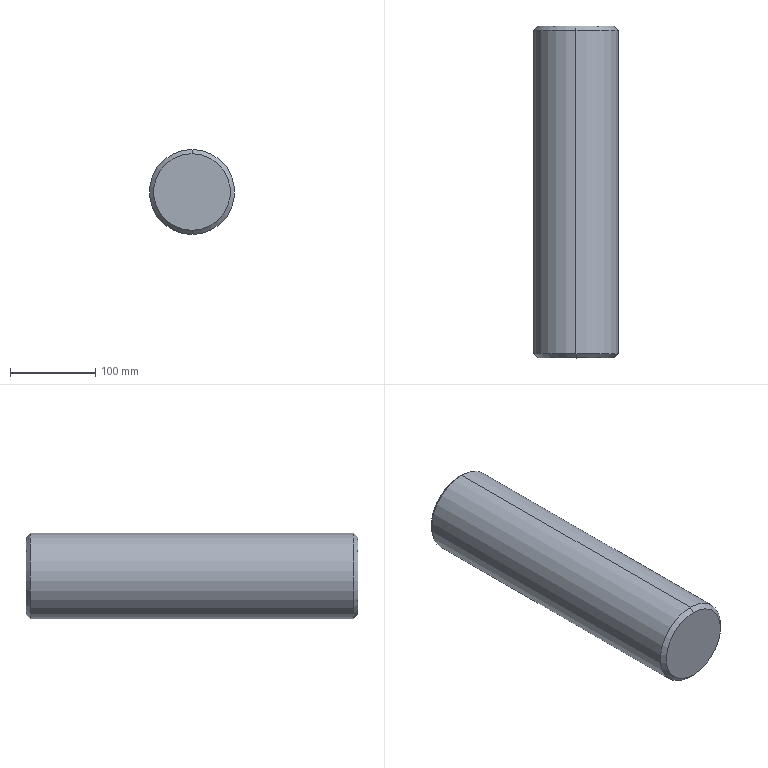Component | SolidWorks | Axis-1 | 1 solid | 8 faces | box 100 x 390 x 100 mm | volume 3055461 mm3 | cone 4 | cylinder 2 | plane 2 | commonest cylinder face diameters 100 x2 | material Plain Carbon Steel
build123d program:
from build123d import *

# Parameters (mm, degrees)
SKETCH1_R           = 50
BOSS_EXTRUDE1_DEPTH = 390
CHAMFER1_SIZE       = 5


with BuildPart() as part:
    # Sketch1 → Boss-Extrude1 (new body)
    with BuildSketch(Plane(origin=(0, 0, 0), x_dir=(0, 0, -1), z_dir=(1, 0, 0))):
        Circle(SKETCH1_R)
    extrude(amount=BOSS_EXTRUDE1_DEPTH)

    # Chamfer1
    chamfer1_edges = [part.edges().sort_by_distance(p)[0] for p in [
        (0, 0, 50),
        (390, 0, 50),
    ]]
    chamfer(chamfer1_edges, length=CHAMFER1_SIZE)


solid = part.part

# Placed as in the assembly
solid = solid.moved(Location((1250.579, 1061.349, 1853.088), (0, 0, 90)))
STEP:
#1=COLOUR_RGB('',0.7922,0.8196,0.9333);
#2=FILL_AREA_STYLE_COLOUR('',#1);
#3=FILL_AREA_STYLE('',(#2));
#4=SURFACE_STYLE_FILL_AREA(#3);
#5=SURFACE_SIDE_STYLE('',(#4));
#6=SURFACE_STYLE_USAGE(.BOTH.,#5);
#7=PRESENTATION_STYLE_ASSIGNMENT((#6));
#8=CARTESIAN_POINT('',(49.235,41.785,74.728));
#9=VERTEX_POINT('',#8);
#10=CARTESIAN_POINT('',(49.235,41.785,71.185));
#11=VERTEX_POINT('',#10);
#12=CARTESIAN_POINT('',(49.235,41.785,72.956));
#13=DIRECTION('',(0.,-1.,0.));
#14=DIRECTION('',(0.,0.,-1.));
#15=AXIS2_PLACEMENT_3D('',#12,#13,#14);
#16=CIRCLE('',#15,1.772);
#17=EDGE_CURVE('',#9,#11,#16,.T.);
#18=ORIENTED_EDGE('',*,*,#17,.F.);
#19=CARTESIAN_POINT('',(49.235,41.982,74.925));
#20=VERTEX_POINT('',#19);
#21=CARTESIAN_POINT('',(49.235,41.982,74.925));
#22=DIRECTION('',(-0.,0.7071,0.7071));
#23=VECTOR('',#22,39.37);
#24=LINE('',#21,#23);
#25=EDGE_CURVE('',#9,#20,#24,.T.);
#26=ORIENTED_EDGE('',*,*,#25,.T.);
#27=CARTESIAN_POINT('',(49.235,41.982,70.988));
#28=VERTEX_POINT('',#27);
#29=CARTESIAN_POINT('',(49.235,41.982,72.956));
#30=DIRECTION('',(-0.,1.,0.));
#31=DIRECTION('',(0.,0.,-1.));
#32=AXIS2_PLACEMENT_3D('',#29,#30,#31);
#33=CIRCLE('',#32,1.969);
#34=EDGE_CURVE('',#28,#20,#33,.T.);
#35=ORIENTED_EDGE('',*,*,#34,.F.);
#36=CARTESIAN_POINT('',(49.235,41.982,70.988));
#37=DIRECTION('',(-0.,0.7071,-0.7071));
#38=VECTOR('',#37,39.37);
#39=LINE('',#36,#38);
#40=EDGE_CURVE('',#11,#28,#39,.T.);
#41=ORIENTED_EDGE('',*,*,#40,.F.);
#42=EDGE_LOOP('',(#18,#26,#35,#41));
#43=FACE_OUTER_BOUND('',#42,.T.);
#44=CARTESIAN_POINT('',(49.235,41.982,72.956));
#45=DIRECTION('',(-0.,1.,0.));
#46=DIRECTION('',(0.,0.,-1.));
#47=AXIS2_PLACEMENT_3D('',#44,#45,#46);
#48=CONICAL_SURFACE('',#47,1.969,0.7854);
#49=ADVANCED_FACE('',(#43),#48,.T.);
#50=CARTESIAN_POINT('',(49.235,57.14,71.185));
#51=VERTEX_POINT('',#50);
#52=CARTESIAN_POINT('',(49.235,57.14,74.728));
#53=VERTEX_POINT('',#52);
#54=CARTESIAN_POINT('',(49.235,57.14,72.956));
#55=DIRECTION('',(-0.,1.,0.));
#56=DIRECTION('',(0.,0.,-1.));
#57=AXIS2_PLACEMENT_3D('',#54,#55,#56);
#58=CIRCLE('',#57,1.772);
#59=EDGE_CURVE('',#51,#53,#58,.T.);
#60=ORIENTED_EDGE('',*,*,#59,.F.);
#61=CARTESIAN_POINT('',(49.235,56.943,70.988));
#62=VERTEX_POINT('',#61);
#63=CARTESIAN_POINT('',(49.235,57.14,71.185));
#64=DIRECTION('',(0.,-0.7071,-0.7071));
#65=VECTOR('',#64,39.37);
#66=LINE('',#63,#65);
#67=EDGE_CURVE('',#51,#62,#66,.T.);
#68=ORIENTED_EDGE('',*,*,#67,.T.);
#69=CARTESIAN_POINT('',(49.235,56.943,74.925));
#70=VERTEX_POINT('',#69);
#71=CARTESIAN_POINT('',(49.235,56.943,72.956));
#72=DIRECTION('',(0.,-1.,0.));
#73=DIRECTION('',(-0.,0.,-1.));
#74=AXIS2_PLACEMENT_3D('',#71,#72,#73);
#75=CIRCLE('',#74,1.969);
#76=EDGE_CURVE('',#70,#62,#75,.T.);
#77=ORIENTED_EDGE('',*,*,#76,.F.);
#78=CARTESIAN_POINT('',(49.235,57.14,74.728));
#79=DIRECTION('',(0.,-0.7071,0.7071));
#80=VECTOR('',#79,39.37);
#81=LINE('',#78,#80);
#82=EDGE_CURVE('',#53,#70,#81,.T.);
#83=ORIENTED_EDGE('',*,*,#82,.F.);
#84=EDGE_LOOP('',(#60,#68,#77,#83));
#85=FACE_OUTER_BOUND('',#84,.T.);
#86=CARTESIAN_POINT('',(49.235,57.14,72.956));
#87=DIRECTION('',(0.,-1.,0.));
#88=DIRECTION('',(0.,0.,1.));
#89=AXIS2_PLACEMENT_3D('',#86,#87,#88);
#90=CONICAL_SURFACE('',#89,1.772,0.7854);
#91=ADVANCED_FACE('',(#85),#90,.T.);
#92=ORIENTED_EDGE('',*,*,#76,.T.);
#93=CARTESIAN_POINT('',(49.235,57.14,70.988));
#94=DIRECTION('',(0.,-1.,0.));
#95=VECTOR('',#94,39.37);
#96=LINE('',#93,#95);
#97=EDGE_CURVE('',#62,#28,#96,.T.);
#98=ORIENTED_EDGE('',*,*,#97,.T.);
#99=ORIENTED_EDGE('',*,*,#34,.T.);
#100=CARTESIAN_POINT('',(49.235,57.14,74.925));
#101=DIRECTION('',(0.,-1.,0.));
#102=VECTOR('',#101,39.37);
#103=LINE('',#100,#102);
#104=EDGE_CURVE('',#70,#20,#103,.T.);
#105=ORIENTED_EDGE('',*,*,#104,.F.);
#106=EDGE_LOOP('',(#92,#98,#99,#105));
#107=FACE_OUTER_BOUND('',#106,.T.);
#108=CARTESIAN_POINT('',(49.235,57.14,72.956));
#109=DIRECTION('',(0.,-1.,0.));
#110=DIRECTION('',(0.,0.,1.));
#111=AXIS2_PLACEMENT_3D('',#108,#109,#110);
#112=CYLINDRICAL_SURFACE('',#111,1.969);
#113=ADVANCED_FACE('',(#107),#112,.T.);
#114=ORIENTED_EDGE('',*,*,#97,.F.);
#115=CARTESIAN_POINT('',(49.235,56.943,72.956));
#116=DIRECTION('',(0.,-1.,0.));
#117=DIRECTION('',(0.,0.,-1.));
#118=AXIS2_PLACEMENT_3D('',#115,#116,#117);
#119=CIRCLE('',#118,1.969);
#120=EDGE_CURVE('',#62,#70,#119,.T.);
#121=ORIENTED_EDGE('',*,*,#120,.T.);
#122=ORIENTED_EDGE('',*,*,#104,.T.);
#123=CARTESIAN_POINT('',(49.235,41.982,72.956));
#124=DIRECTION('',(-0.,1.,0.));
#125=DIRECTION('',(0.,0.,-1.));
#126=AXIS2_PLACEMENT_3D('',#123,#124,#125);
#127=CIRCLE('',#126,1.969);
#128=EDGE_CURVE('',#20,#28,#127,.T.);
#129=ORIENTED_EDGE('',*,*,#128,.T.);
#130=EDGE_LOOP('',(#114,#121,#122,#129));
#131=FACE_OUTER_BOUND('',#130,.T.);
#132=CARTESIAN_POINT('',(49.235,57.14,72.956));
#133=DIRECTION('',(0.,-1.,0.));
#134=DIRECTION('',(0.,0.,1.));
#135=AXIS2_PLACEMENT_3D('',#132,#133,#134);
#136=CYLINDRICAL_SURFACE('',#135,1.969);
#137=ADVANCED_FACE('',(#131),#136,.T.);
#138=CARTESIAN_POINT('',(49.235,57.14,72.956));
#139=DIRECTION('',(-0.,1.,0.));
#140=DIRECTION('',(0.,0.,-1.));
#141=AXIS2_PLACEMENT_3D('',#138,#139,#140);
#142=CIRCLE('',#141,1.772);
#143=EDGE_CURVE('',#53,#51,#142,.T.);
#144=ORIENTED_EDGE('',*,*,#143,.T.);
#145=ORIENTED_EDGE('',*,*,#59,.T.);
#146=EDGE_LOOP('',(#144,#145));
#147=FACE_OUTER_BOUND('',#146,.T.);
#148=CARTESIAN_POINT('',(49.235,57.14,72.956));
#149=DIRECTION('',(-0.,1.,0.));
#150=DIRECTION('',(0.,0.,-1.));
#151=AXIS2_PLACEMENT_3D('',#148,#149,#150);
#152=PLANE('',#151);
#153=ADVANCED_FACE('',(#147),#152,.T.);
#154=CARTESIAN_POINT('',(49.235,41.785,72.956));
#155=DIRECTION('',(0.,-1.,0.));
#156=DIRECTION('',(0.,0.,-1.));
#157=AXIS2_PLACEMENT_3D('',#154,#155,#156);
#158=CIRCLE('',#157,1.772);
#159=EDGE_CURVE('',#11,#9,#158,.T.);
#160=ORIENTED_EDGE('',*,*,#159,.T.);
#161=ORIENTED_EDGE('',*,*,#17,.T.);
#162=EDGE_LOOP('',(#160,#161));
#163=FACE_OUTER_BOUND('',#162,.T.);
#164=CARTESIAN_POINT('',(49.235,41.785,72.956));
#165=DIRECTION('',(-0.,1.,0.));
#166=DIRECTION('',(0.,0.,-1.));
#167=AXIS2_PLACEMENT_3D('',#164,#165,#166);
#168=PLANE('',#167);
#169=ADVANCED_FACE('',(#163),#168,.F.);
#170=ORIENTED_EDGE('',*,*,#67,.F.);
#171=ORIENTED_EDGE('',*,*,#143,.F.);
#172=ORIENTED_EDGE('',*,*,#82,.T.);
#173=ORIENTED_EDGE('',*,*,#120,.F.);
#174=EDGE_LOOP('',(#170,#171,#172,#173));
#175=FACE_OUTER_BOUND('',#174,.T.);
#176=CARTESIAN_POINT('',(49.235,57.14,72.956));
#177=DIRECTION('',(0.,-1.,0.));
#178=DIRECTION('',(0.,0.,1.));
#179=AXIS2_PLACEMENT_3D('',#176,#177,#178);
#180=CONICAL_SURFACE('',#179,1.772,0.7854);
#181=ADVANCED_FACE('',(#175),#180,.T.);
#182=ORIENTED_EDGE('',*,*,#25,.F.);
#183=ORIENTED_EDGE('',*,*,#159,.F.);
#184=ORIENTED_EDGE('',*,*,#40,.T.);
#185=ORIENTED_EDGE('',*,*,#128,.F.);
#186=EDGE_LOOP('',(#182,#183,#184,#185));
#187=FACE_OUTER_BOUND('',#186,.T.);
#188=CARTESIAN_POINT('',(49.235,41.982,72.956));
#189=DIRECTION('',(-0.,1.,0.));
#190=DIRECTION('',(0.,0.,-1.));
#191=AXIS2_PLACEMENT_3D('',#188,#189,#190);
#192=CONICAL_SURFACE('',#191,1.969,0.7854);
#193=ADVANCED_FACE('',(#187),#192,.T.);
#194=CLOSED_SHELL('',(#49,#91,#113,#137,#153,#169,#181,#193));
#195=MANIFOLD_SOLID_BREP('',#194);
#196=STYLED_ITEM('',(#7),#195);
#197=(LENGTH_UNIT()NAMED_UNIT(*)SI_UNIT($,.METRE.));
#198=LENGTH_MEASURE_WITH_UNIT(LENGTH_MEASURE(0.0254),#197);
#199=DIMENSIONAL_EXPONENTS(1.,0.,0.,0.,0.,0.,0.);
#200=(CONVERSION_BASED_UNIT('',#198)LENGTH_UNIT()NAMED_UNIT(#199));
#201=UNCERTAINTY_MEASURE_WITH_UNIT(LENGTH_MEASURE(0.00001),#200,'','');
#202=(NAMED_UNIT(*)PLANE_ANGLE_UNIT()SI_UNIT($,.RADIAN.));
#203=(NAMED_UNIT(*)SI_UNIT($,.STERADIAN.)SOLID_ANGLE_UNIT());
#204=(GEOMETRIC_REPRESENTATION_CONTEXT(3)GLOBAL_UNCERTAINTY_ASSIGNED_CONTEXT((#201))GLOBAL_UNIT_ASSIGNED_CONTEXT((#200,#202,#203))REPRESENTATION_CONTEXT('',''));
#205=MECHANICAL_DESIGN_GEOMETRIC_PRESENTATION_REPRESENTATION('',(#196),#204);
#206=CARTESIAN_POINT('',(0.,0.,0.));
#207=DIRECTION('',(0.,0.,1.));
#208=DIRECTION('',(1.,0.,0.));
#209=AXIS2_PLACEMENT_3D('',#206,#207,#208);
#210=(LENGTH_UNIT()NAMED_UNIT(*)SI_UNIT($,.METRE.));
#211=LENGTH_MEASURE_WITH_UNIT(LENGTH_MEASURE(0.0254),#210);
#212=DIMENSIONAL_EXPONENTS(1.,0.,0.,0.,0.,0.,0.);
#213=(CONVERSION_BASED_UNIT('',#211)LENGTH_UNIT()NAMED_UNIT(#212));
#214=UNCERTAINTY_MEASURE_WITH_UNIT(LENGTH_MEASURE(0.00001),#213,'','');
#215=(NAMED_UNIT(*)PLANE_ANGLE_UNIT()SI_UNIT($,.RADIAN.));
#216=(NAMED_UNIT(*)SI_UNIT($,.STERADIAN.)SOLID_ANGLE_UNIT());
#217=(GEOMETRIC_REPRESENTATION_CONTEXT(3)GLOBAL_UNCERTAINTY_ASSIGNED_CONTEXT((#214))GLOBAL_UNIT_ASSIGNED_CONTEXT((#213,#215,#216))REPRESENTATION_CONTEXT('',''));
#218=ADVANCED_BREP_SHAPE_REPRESENTATION('',(#195,#209),#217);
#219=PRESENTATION_LAYER_ASSIGNMENT('','',(#196));